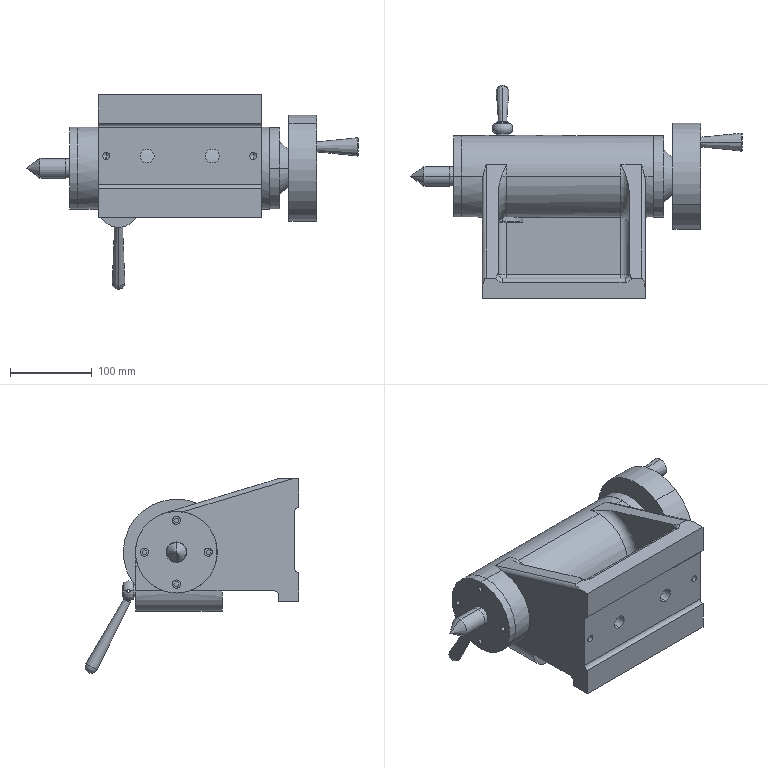Assembly | SolidWorks | mm | 24 component files | 24 solids | 412 faces | box 406.58 x 261.83 x 238.27 mm | volume 3779107 mm3 | plane 180 | cylinder 176 | cone 44 | torus 12 | commonest cylinder face diameters 10 x45 6.8 x32 20 x12 50 x11 25 x8 8.5 x8 62 x8 100 x8
Bill of materials:
FrontEndCap | 1 |  | Flat circular disc flange with a raised concentric cylindrical boss on one face, a central through bore, and four equally spaced through holes on a circle between the boss and the outer rim.
Handle_2 | 1 |  | Solid body of revolution: a short small-diameter cylindrical spigot at one end, joined at a step to a long conical frustum that widens toward a flat, large-diameter end face with a small edge chamfer or bevel.
Handle | 1 |  | L-shaped lever or crank-like form. A straight cylindrical rod ends in a rounded, roughly spherical hub with a collar. A second arm comes off the hub at an obtuse angle, tapers toward its end, and finishes in a rounded tip. The hub has a small cross hole.
Handwheel | 1 |  | Thick circular disc with a central through hole and a smaller off-center hole near the rim on one face.
Key5x5x16 | 1 |  | Plain rectangular block with flat faces and sharp edges. It looks roughly square in one view and has no visible holes or features.
LiveCenter | 1 |  | Long, slender cylindrical pin with a conical pointed tip at one end and a flat end face at the other. The body may taper slightly along its length.
LowerBushing | 1 |  | Thick-walled cylindrical sleeve or bushing with a central through bore. Its length is about equal to its outer diameter.
NutM12 | 1 |  | Hexagonal nut-like body with a central round through bore and chamfered corners on both faces, which leave curved arc boundaries on the flats.
Part4^LatheTailstock | 1 |  | Cylindrical tube or spacer, several diameters long, with a central through bore and flat ends.
RearEndCap | 1 |  | Circular flange with a tapered conical hub rising from one face, a central through bore, and four equally spaced through holes on a circle outside the hub.
ScrewM10X20 | 1 |  | Stepped cylindrical shaft: a smaller-diameter section joined at a shoulder to a larger-diameter section. The larger section has a slot cut axially into its end, and it may have a slight further diameter step near that end.
ScrewM8X20 | 8 |  | Stepped solid cylindrical pin: a short larger-diameter head section and a longer smaller-diameter shank, both with flat ends.
ScrewRod | 1 |  | Stepped, rotationally symmetric shaft. A long plain cylindrical section leads to a thin integral disc-shaped collar, followed by several shorter sections that get smaller in diameter, ending in a small pilot end. One of the stepped sections has a shallow slot like a keyway.
TailstockBody | 1 |  | Block-shaped housing with a large cylindrical through-bore along its length. Round bosses stick out from each end face, and each has a pattern of small holes around the bore. A rectangular window in one face exposes the bore. The side profile is tapered, and the base has notches and steps.
UpperBushing | 1 |  | Thick-walled plain cylindrical tube or sleeve with a concentric through-bore and flat, square ends.
Washer | 1 |  | Thin flat annular ring like a washer, with a rectangular cross-section, a large central opening and a narrow radial width.
Washer12 | 1 |  | Thin flat annular ring like a washer, with a rectangular cross-section, a large central opening and a narrow radial width.
Mates:
1. concentric | TailstockBody-1 face at (-401, 150, -15) dir (1, 0, 0) r 31 | Part4^LatheTailstock-1 face at (-81.446, 150, -15) dir (1, 0, 0) r 31
2. concentric | LiveCenter-2 face at (-8.319, 150, -15) dir (1, 0, 0) r 17.453 | Part4^LatheTailstock-1 face at (-81.446, 150, -15) dir (1, 0, 0) r 12
3. concentric | ScrewRod-1 face at (18.554, 150, -15) dir (-1, 0, 0) r 12 | Part4^LatheTailstock-1 face at (-81.446, 150, -15) dir (1, 0, 0) r 12
4. coincident | ScrewRod-1 face at (18.554, 150, -15) dir (-1, 0, 0) | Part4^LatheTailstock-1 face at (18.554, 150, -15) dir (-1, 0, 0)
5. coincident | TailstockBody-1 face at (110, 0, 0) dir (1, 0, 0) | RearEndCap-1 face at (110, 150, -65) dir (-1, 0, 0)
6. concentric | ScrewRod-1 face at (18.554, 150, -15) dir (-1, 0, 0) r 10 | RearEndCap-1 face at (154.24, 150, -15) dir (1, 0, 0) r 11
7. concentric | TailstockBody-1 face at (-125, 150, -15) dir (1, 0, 0) r 50 | Washer-1 face at (117.554, 150, -15) dir (-1, 0, 0) r 31
8. coincident | RearEndCap-1 face at (117.554, 150, -15) dir (-1, 0, 0) | Washer-1 edge at (117.554, 150, -15) dir (1, 0, 0) r 25
9. coincident | ScrewRod-1 face at (112.554, 137.212, -36.482) dir (1, 0, 0) | Washer-1 face at (112.554, 150, -15) dir (-1, 0, 0)
10. concentric | UpperBushing-1 face at (-75, 170.565, -62.5) dir (0, 1, 0) r 12.5 | LowerBushing-1 face at (-75, 150.512, -62.5) dir (0, -1, 0) r 12.5
11. concentric | TailstockBody-1 edge at (-75, 200, -62.5) dir (0, 1, 0) r 12.5 | UpperBushing-1 face at (-75, 170.565, -62.5) dir (0, 1, 0) r 12.5
12. concentric | TailstockBody-1 face at (-30.009, 200, -15) dir (0, 1, 0) r 4.25 | ScrewM10X20-1 edge at (-30.009, 200, -15) dir (0, 1, 0) r 4.25
13. tangent | TailstockBody-1 face at (-125, 150, -15) dir (1, 0, 0) r 50 | ScrewM10X20-1 face at (-30.009, 200, -15) dir (0, 1, 0)
14. concentric | FrontEndCap-1 edge at (-135, 189, -15) dir (-1, 0, 0) r 5 | ScrewM8X20-1 face at (-135, 189, -15) dir (1, 0, 0) r 5
15. concentric | LiveCenter-2 face at (-188.319, 150, -15) dir (-1, 0, 0) r 12 | FrontEndCap-1 face at (-186.015, 150, -15) dir (-1, 0, 0) r 50
16. coincident | TailstockBody-1 edge at (-125, 150, -15) dir (1, 0, 0) r 50 | FrontEndCap-1 edge at (-125, 150, -15) dir (-1, 0, 0) r 50
17. coincident | FrontEndCap-1 face at (-135, 162.567, -15) dir (-1, 0, 0) | ScrewM8X20-1 face at (-135, 189, -15) dir (-1, 0, 0)
18. concentric | FrontEndCap-1 edge at (-125, 189, -15) dir (-1, 0, 0) r 5 | ScrewM8X20-1 face at (-104, 189, -15) dir (-1, 0, 0) r 3.4
19. concentric | TailstockBody-1 face at (-125, 189, -15) dir (-1, 0, 0) r 3.4 | ScrewM8X20-1 face at (-135, 189, -15) dir (1, 0, 0) r 5
20. concentric | RearEndCap-1 edge at (122.554, 189, -15) dir (-1, 0, 0) r 5 | ScrewM8X20-5 edge at (122.554, 189, -15) dir (1, 0, 0) r 5
21. concentric | ScrewRod-1 face at (18.554, 150, -15) dir (-1, 0, 0) r 10 | Washer12-1 face at (151.052, 150, -15) dir (-1, 0, 0) r 10
22. concentric | TailstockBody-1 face at (-125, 150, -15) dir (1, 0, 0) r 50 | Handwheel-1 face at (167.63, 150, -15) dir (-1, 0, 0) r 65
23. coincident | RearEndCap-1 edge at (133.63, 150, -15) dir (1, 0, 0) r 22.896 | Handwheel-1 face at (133.63, 150, -15) dir (-1, 0, 0)
24. concentric | Handwheel-1 face at (159.63, 191.81, 11.106) dir (1, 0, 0) r 5 | Handle_2-1 face at (159.63, 191.81, 11.106) dir (1, 0, 0) r 5
25. coincident | Handwheel-1 face at (167.63, 150, -15) dir (1, 0, 0) | Handle_2-1 face at (167.63, 191.81, 11.106) dir (-1, 0, 0)
26. concentric | ScrewRod-1 face at (18.554, 150, -15) dir (-1, 0, 0) r 6 | NutM12-1 face at (158.052, 150, -15) dir (-1, 0, 0) r 6
27. coincident | Washer12-1 face at (151.052, 150, -15) dir (1, 0, 0) | NutM12-1 face at (151.052, 3.425, 20.224) dir (-1, 0, 0)
28. parallel | ScrewRod-1 face at (133.654, 152.545, -13.411) dir (0, -0.8482, -0.5296) | Handwheel-1 face at (133.63, 146.076, -3.132) dir (0, -0.8482, -0.5296)
29. parallel | Handwheel-1 face at (133.63, 146.076, -3.132) dir (0, -0.8482, -0.5296) | Key5x5x16-2 face at (143.654, 147.482, -5.326) dir (0, 0.8482, 0.5296)
30. coincident | ScrewRod-1 edge at (133.654, 148.889, -7.556) dir (1, 0, 0) | Key5x5x16-2 edge at (143.654, 148.889, -7.556) dir (-1, 0, 0)
31. coincident | ScrewRod-1 face at (133.654, 150, -15) dir (1, 0, 0) | Key5x5x16-2 face at (133.654, 14.855, -81.716) dir (-1, 0, 0)